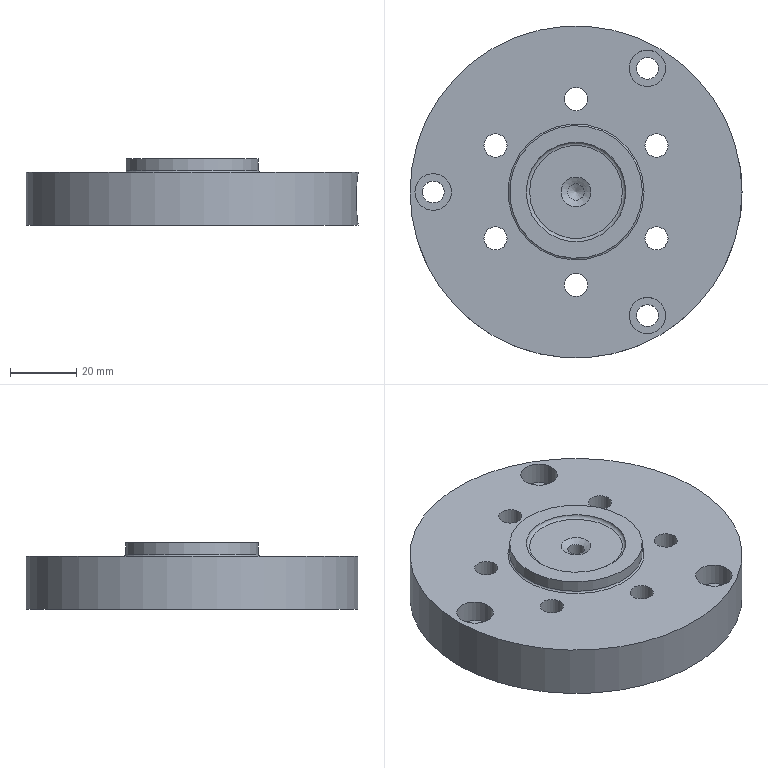Component | NX | END_CAP | 1 solid | 45 faces | volume 115368 mm3 | cylinder 24 | plane 15 | cone 3 | torus 3 | commonest cylinder face diameters 11 x9 7 x6 6.6 x3 5 x2 100 x1 40 x1 9.728 x1 15 x1